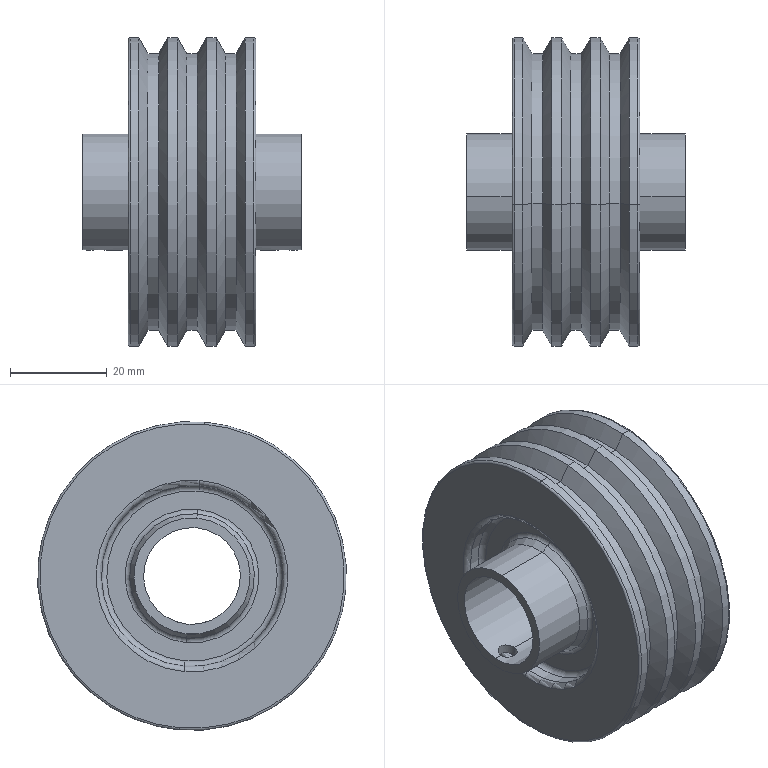Component | SolidWorks | Poly-VPulley-1 | 1 solid | 66 faces | box 45.22 x 63.8 x 63.8 mm | volume 65367 mm3 | cylinder 28 | cone 16 | torus 16 | plane 6 | commonest cylinder face diameters 63.8 x8 57.2 x6 4 x4 24 x4 37.4 x4 20 x2
build123d program:
from build123d import *

# Parameters (mm, degrees)
SCALE1_SCALE                    = 0.22
SKETCH1_2_R                     = 10
CUT_EXTRUDE1_DEPTH              = 52.975
SKETCH2_R                       = 12
SKETCH2_R_2                     = 10
BOSS_EXTRUDE1_DEPTH             = 10
BOSS_EXTRUDE1_DIRECTION_2_REACH = 53.975
SKETCH3_R                       = 2
CUT_EXTRUDE2_DEPTH              = 10


with BuildPart() as part:
    # Sketch1 → Revolve Boss (revolve)
    with BuildSketch(Plane(origin=(0, 0, 0), x_dir=(0, 0, -1), z_dir=(1, 0, 0)), mode=Mode.PRIVATE) as revolve_boss_sk:
        with BuildLine():
            Line((-60, 90), (-60, 143))
            ThreePointArc((-60, 143), (-59.414, 144.414), (-58, 145))
            Line((-58, 145), (-50, 145))
            Line((-50, 145), (-41.34, 130))
            Line((-41.34, 130), (-31.34, 130))
            Line((-31.34, 130), (-22.679, 145))
            Line((-22.679, 145), (-13.66, 145))
            Line((-13.66, 145), (-5, 130))
            Line((-5, 130), (5, 130))
            Line((5, 130), (13.66, 145))
            Line((13.66, 145), (22.679, 145))
            Line((22.679, 145), (31.34, 130))
            Line((31.34, 130), (41.34, 130))
            Line((41.34, 130), (50, 145))
            Line((50, 145), (58, 145))
            ThreePointArc((58, 145), (59.414, 144.414), (60, 143))
            Line((60, 143), (60, 90))
            ThreePointArc((60, 90), (58.536, 86.464), (55, 85))
            Line((55, 85), (45, 85))
            ThreePointArc((45, 85), (41.464, 83.536), (40, 80))
            Line((40, 80), (40, 62.887))
            ThreePointArc((40, 62.887), (40.67, 60.387), (42.5, 58.557))
            Line((42.5, 58.557), (54.821, 51.443))
            ThreePointArc((54.821, 51.443), (56.651, 49.613), (57.321, 47.113))
            Line((57.321, 47.113), (57.321, 25))
            Line((57.321, 25), (-57.321, 25))
            Line((-57.321, 25), (-57.321, 47.113))
            ThreePointArc((-57.321, 47.113), (-56.651, 49.613), (-54.821, 51.443))
            Line((-54.821, 51.443), (-42.5, 58.557))
            ThreePointArc((-42.5, 58.557), (-40.67, 60.387), (-40, 62.887))
            Line((-40, 62.887), (-40, 80))
            ThreePointArc((-40, 80), (-41.464, 83.536), (-45, 85))
            Line((-45, 85), (-55, 85))
            ThreePointArc((-55, 85), (-58.536, 86.464), (-60, 90))
        make_face()
    revolve(revolve_boss_sk.sketch.rotate(Axis((0, 0, 0), (0, 0, -1)), 90), axis=Axis((0, 0, 0), (0, 0, -1)))


with BuildPart() as part_1:
    # Scale1: scaled about (0, 0, 0)
    add(part.part.scale(SCALE1_SCALE))

    # Sketch1_2 → Cut-Extrude1 (cut, through all)
    with BuildSketch(Plane.XY.offset(12.611)):
        Circle(SKETCH1_2_R)
    extrude(amount=-CUT_EXTRUDE1_DEPTH, mode=Mode.SUBTRACT)

    # Sketch2 → Boss-Extrude1 (add)
    with BuildSketch(Plane(origin=(0, 0, -12.611), x_dir=(-1, 0, 0), z_dir=(0, 0, -1))):
        with Locations(Location((0, 0, 0), (0, 0, 180))):
            Circle(SKETCH2_R)
        with Locations(Location((0, 0, 0), (0, 0, 180))):
            Circle(SKETCH2_R_2, mode=Mode.SUBTRACT)
    boss_extrude1 = extrude(amount=BOSS_EXTRUDE1_DEPTH)

    # Sketch2 → Boss-Extrude1 direction 2 (add, up to next)
    with BuildSketch(Plane(origin=(0, 0, -12.611), x_dir=(-1, 0, 0), z_dir=(0, 0, -1)), mode=Mode.PRIVATE) as boss_extrude1_direction_2_sk1:
        with Locations(Location((0, 0, 0), (0, 0, 180))):
            Circle(SKETCH2_R)
        with Locations(Location((0, 0, 0), (0, 0, 180))):
            Circle(SKETCH2_R_2, mode=Mode.SUBTRACT)
    boss_extrude1_direction_2_tool1 = extrude(boss_extrude1_direction_2_sk1.sketch, amount=-BOSS_EXTRUDE1_DIRECTION_2_REACH, mode=Mode.PRIVATE) - part_1.part
    boss_extrude1_direction_2 = boss_extrude1_direction_2_tool1.solids().sort_by_distance((-11.661, 0, -12.611))[0]
    add(boss_extrude1_direction_2)

    # Sketch3 → Cut-Extrude2 (cut)
    with BuildSketch(Plane.ZY.offset(12)):
        with Locations((-19.111, 0)):
            Circle(SKETCH3_R)
    cut_extrude2 = extrude(amount=-CUT_EXTRUDE2_DEPTH, mode=Mode.SUBTRACT)

    # Mirror1: Boss-Extrude1, Boss-Extrude1 direction 2, Cut-Extrude2 across plane
    add(boss_extrude1.mirror(Plane(origin=(0, 0, 0), x_dir=(1, 0, 0), z_dir=(0, 0, -1))))
    add(boss_extrude1_direction_2.mirror(Plane(origin=(0, 0, 0), x_dir=(1, 0, 0), z_dir=(0, 0, -1))))
    add(cut_extrude2.mirror(Plane(origin=(0, 0, 0), x_dir=(1, 0, 0), z_dir=(0, 0, -1))), mode=Mode.SUBTRACT)


solid = part_1.part

# Placed as in the assembly
solid = solid.moved(Location((28.24, 34.1, 498.836), (90.714, -90, 85.878)))